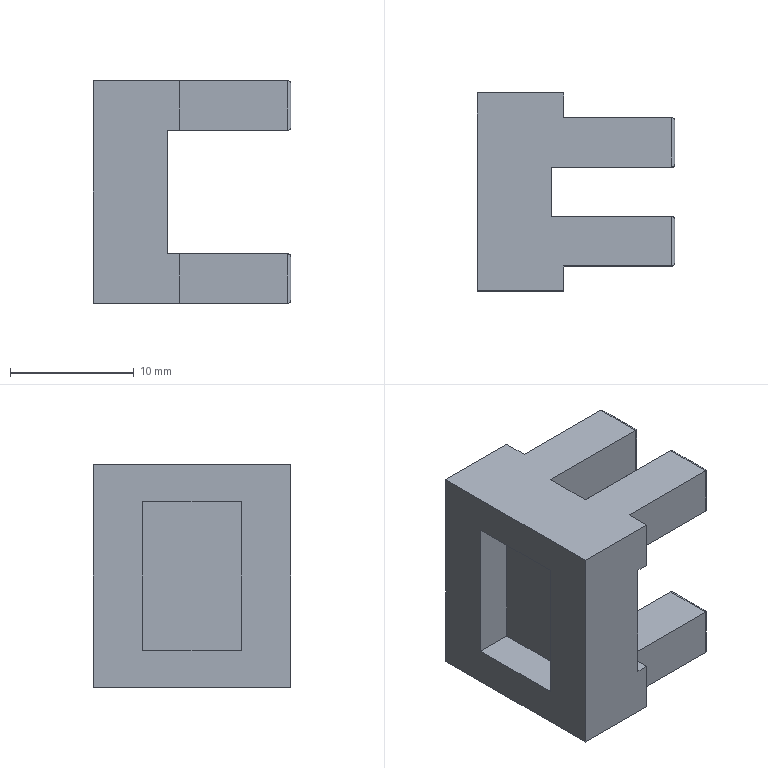Component | NX | 22A__27_2 | 1 solid | 47 faces | volume 2111 mm3 | plane 31 | cylinder 16 | commonest cylinder face diameters 0.5 x16